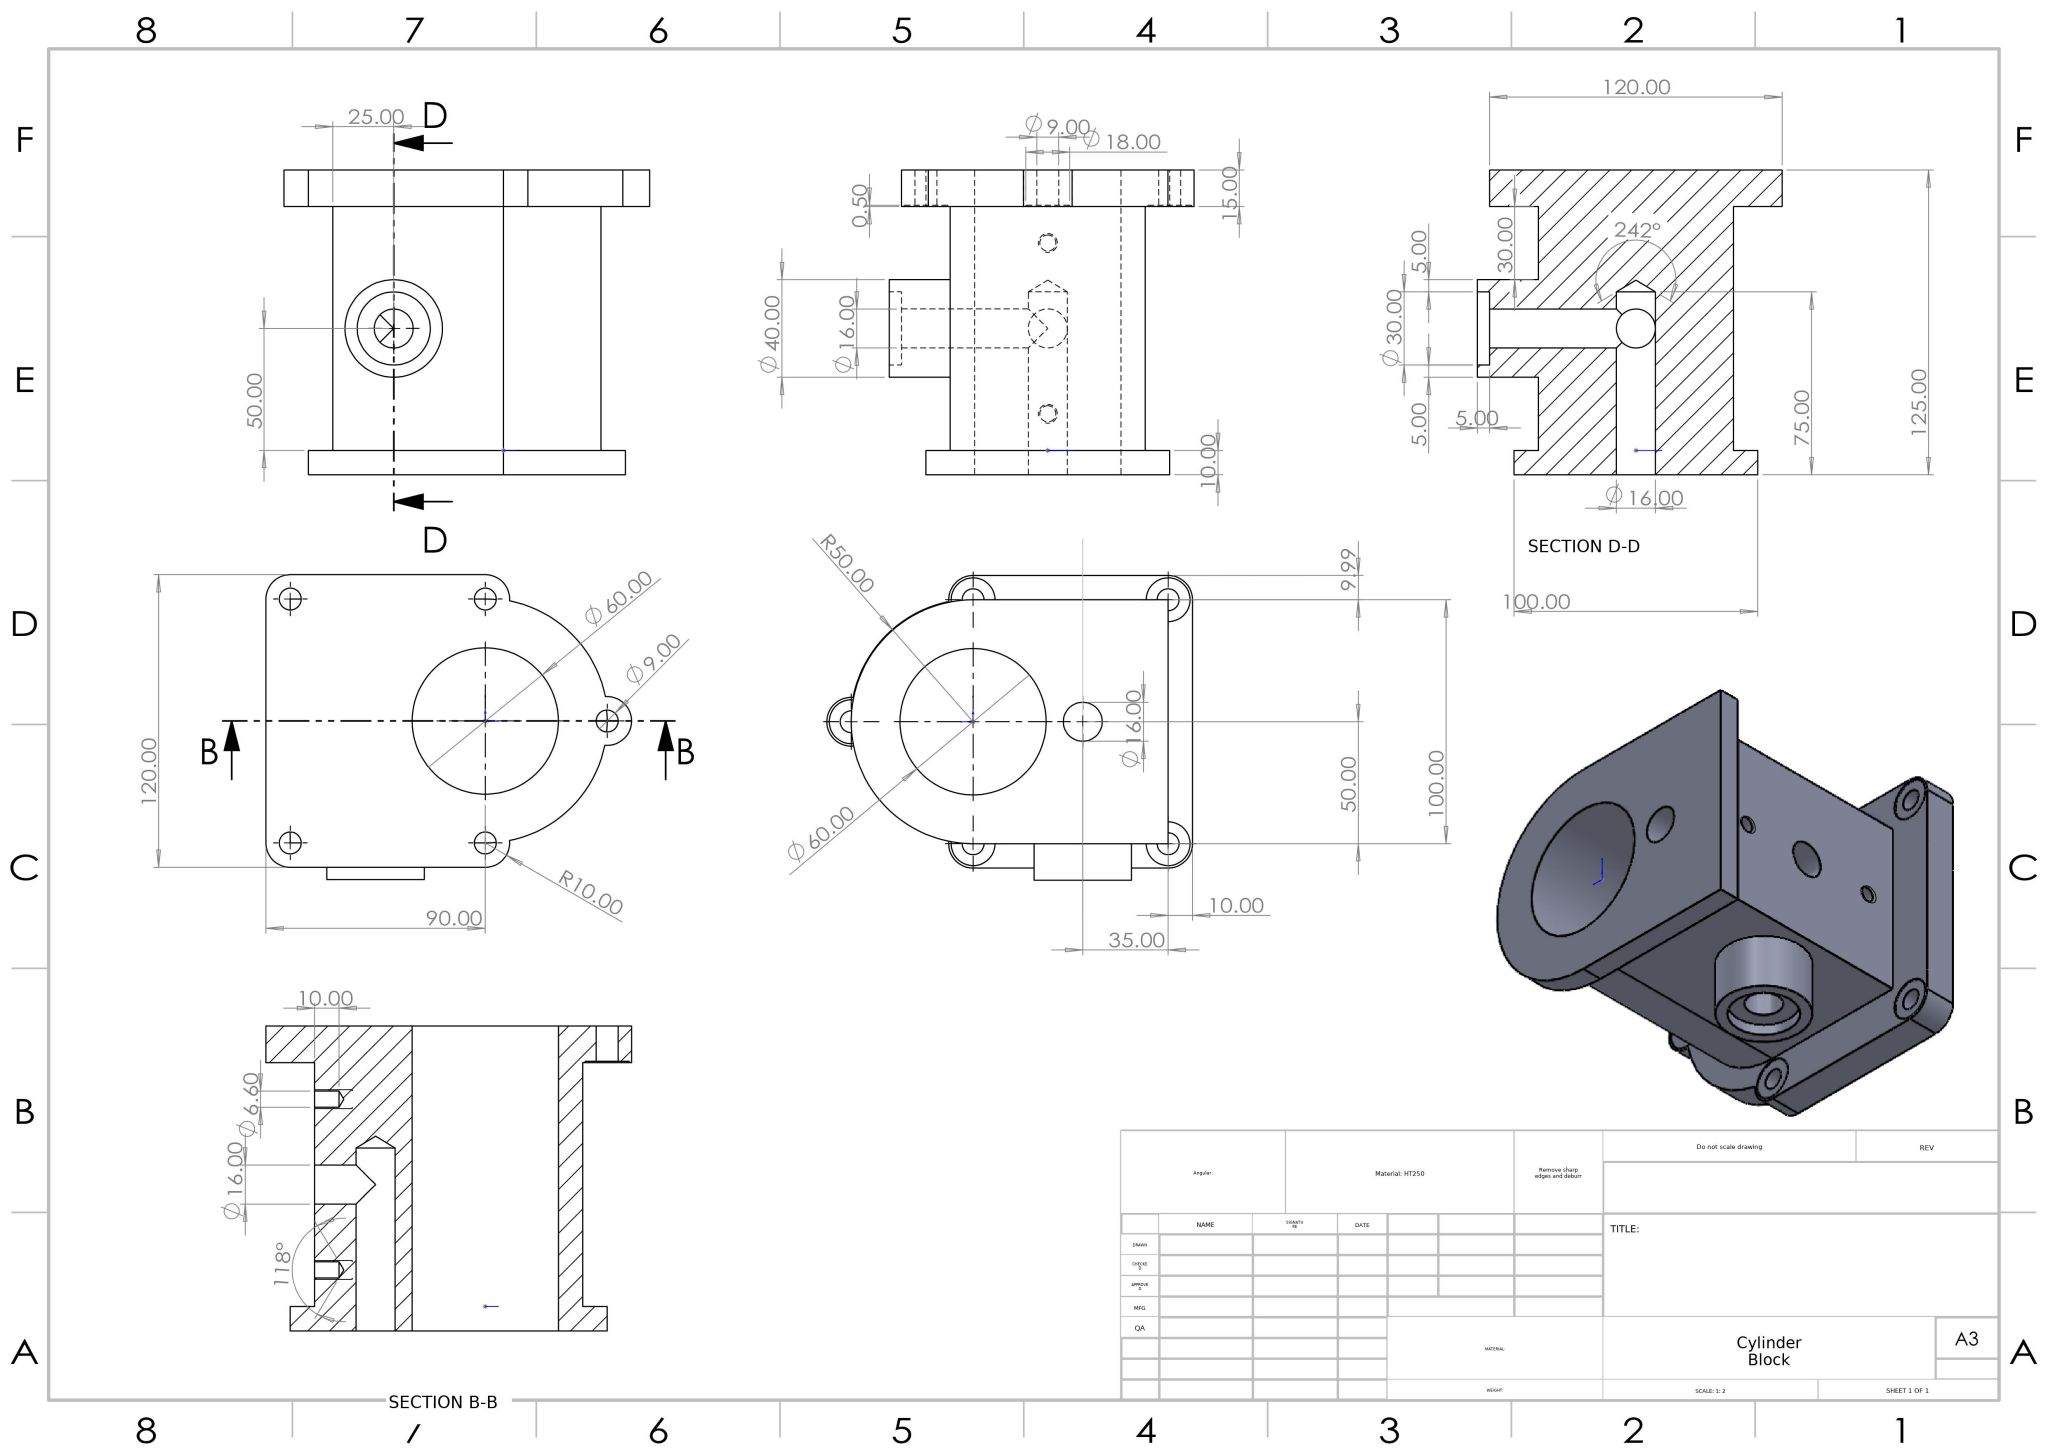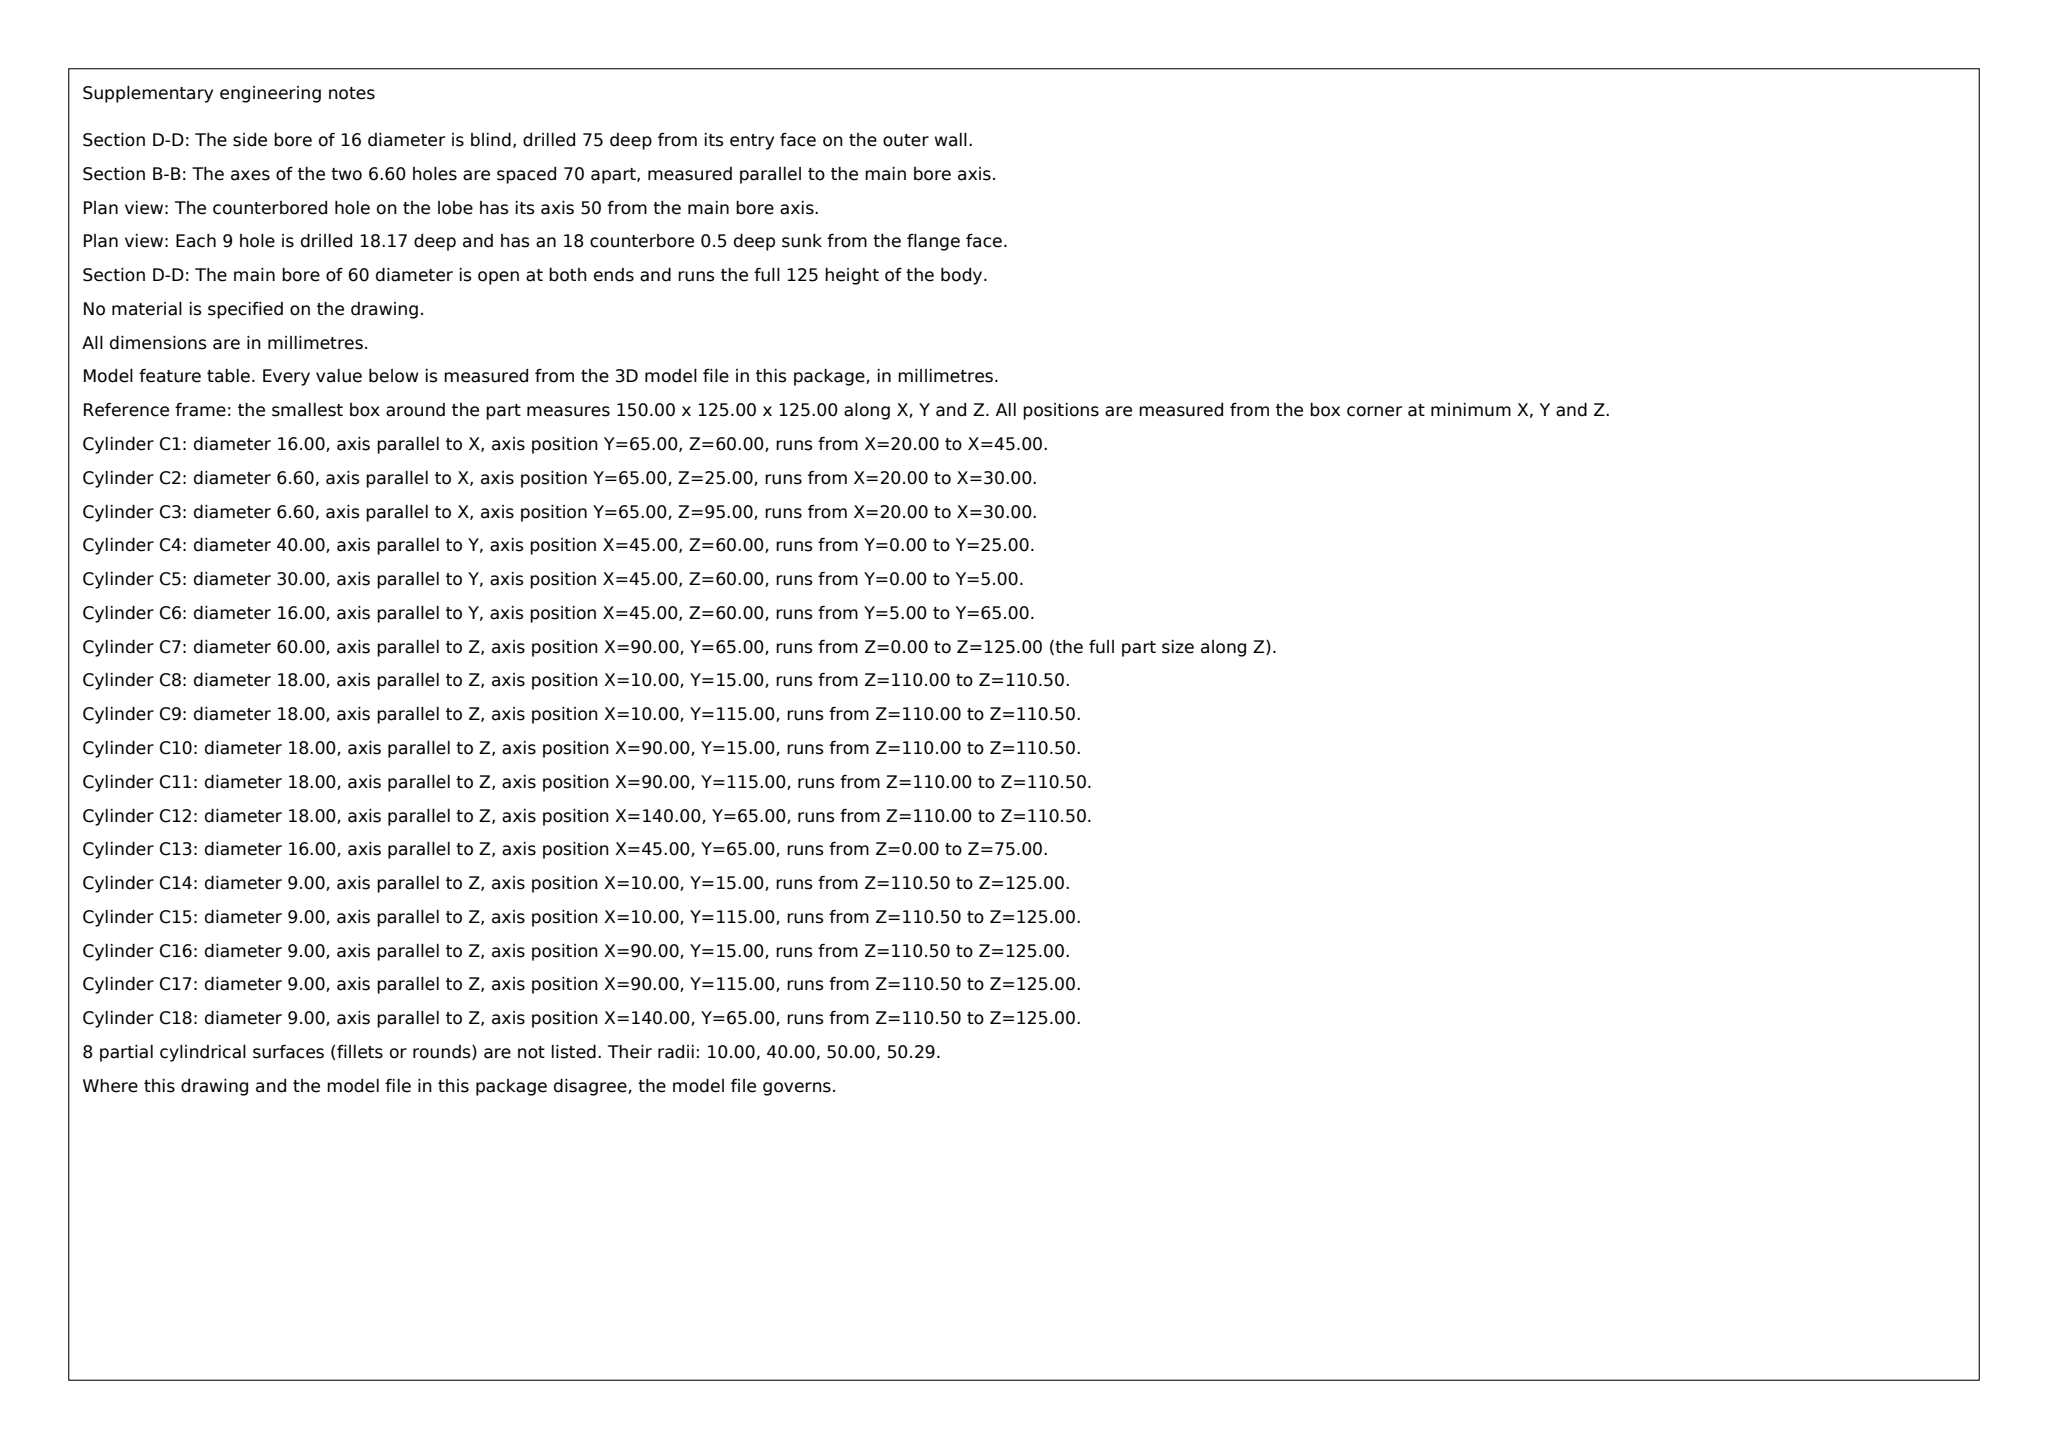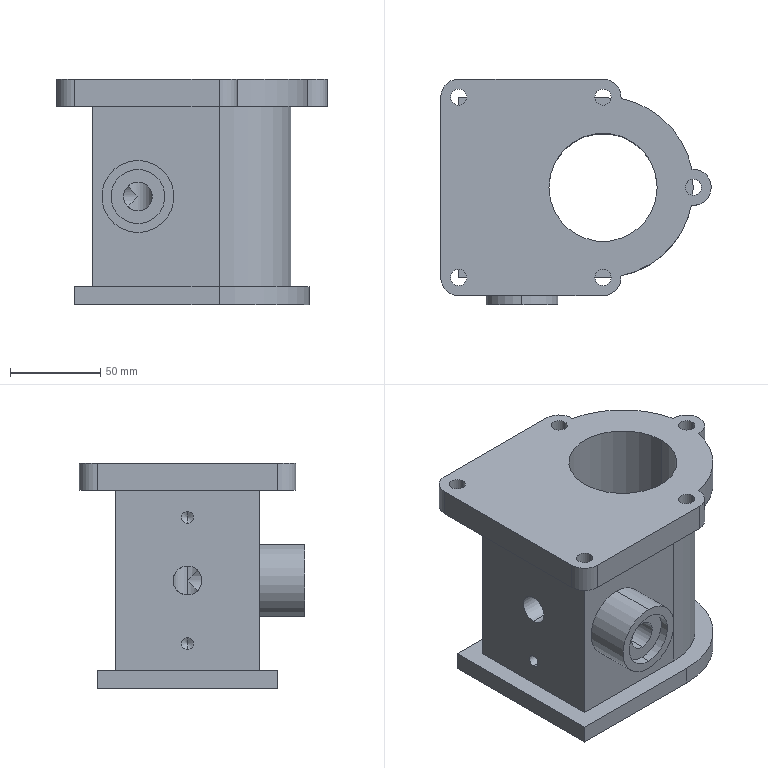Part | SolidWorks | mm | 1 solid | 73 faces | box 150 x 125 x 125 mm | volume 794820 mm3 | cylinder 47 | plane 20 | cone 6 | commonest cylinder face diameters 18 x10 9 x10 16 x7 20 x5 6.6 x4 100 x3 30 x2 40 x2
Drawing notes:
CENTRAL BODY OD Ø80, 100 LG BTWN Ø100 FLANGES | from the solid: cyl [80,"z",[90,65],100] between Ø100 flanges at z0-10 and z110-125
4X Ø6.60 DP 10 (118° PT): CL 25 & 95 FROM BASE, SECT B-B | from the solid: cyls [6.6,"x",[null,65,25],10,2] and [6.6,"x",[null,65,95],10,2]; cones 118°/6.6
SECT B-B: Ø16 BLIND HOLE DP 25 FROM O/S FACE, 118° PT | from the solid: cyl [16,'x',[null,65,60],25.0] with cone 118°, ref_dia 16
ARM Ø16 BORE DP 60 FROM Ø40/Ø30 BOSS END FACE | from the solid: cyl [16,'y',[45,null,60],60.0]; Ø40 L25 & Ø30 L5 boss on same axis
4X Ø6.60 DP 10 118° PT ALL ON CL B-B (Y=65), 2 EA AT 25 & 95 | from the solid: cyls [6.6,'x',[null,65,25],10]x2 and [6.6,'x',[null,65,95],10]x2; 4 cones 118° ref 6.6
SIDE LUG: Ø9 THRU ON Ø20 BOSS, Ø18 SPOTFACE DP 0.50; LUG AXIS AT X=140 FROM PLATE O/S FACE (X=0), Y=65 (PART C/L) | from the solid: cylinders dia 9 (L14.5), dia 18 (L0.5) and dia 20 (L15), axis z, pos [140.0, 65.0]
OVERALL ENVELOPE 150 (X) X 125 (Y) X 125 (Z); X=150 MEASURED FROM PLATE O/S FACE TO SIDE-LUG BOSS O/S | from the solid: bbox_xyz [150.0, 125.0, 125.0]
ARM BOSS: Ø30 X 5 LG FROM END FACE Y=0, THEN Ø40 X 25 LG (ARM PROJECTS 30 TOTAL FROM Y=0); ARM AXIS X=45, Z=60 | from the solid: cylinders dia 30 axis y [45.0,60.0] L5.0 and dia 40 axis y [45.0,60.0] L25.0; planes y=0.0, y=5.0, y=25.0
VERTICAL Ø16 BLIND HOLE DP 75 FROM BASE (Z=0), 118° PT, AXIS AT X=45, Y=65 | from the solid: cylinder dia 16 axis z pos [45.0,65.0] length 75.0; cones 118.0 ref_dia 16.0
4X Ø6.60 DP 10, 118° PT: holes on part C/L Y=65 at Z=25 & 95, axes parallel to X, drilled DP 10 from plate O/S face X=0. | from the solid: cylinders [6.6,"x",[null,65,25],10,2] and [6.6,"x",[null,65,95],10,2]; axis_plane x=0; cones 118° ref dia 6.6 (4)
SIDE LUG: Ø9 THRU on Ø20 boss (boss 15 LG), Ø18 SPOTFACE DP 0.50; lug axis at X=140 from plate O/S face (X=0) and Y=65 (part C/L). | from the solid: cylinders [9.0,"z",[140,65,null],14.5,2], [18.0,"z",[140,65,null],0.5,2], [20.0,"z",[140,65,null],15.0,1]
OVERALL ENVELOPE 150 (X) X 125 (Y) X 125 (Z); X=150 from plate O/S face (X=0) to side-lug boss O/S. | from the solid: bbox_xyz [150.0,125.0,125.0]
ARM BOSS: Ø30 X 5 LG from end face Y=0, then Ø40 X 25 LG (arm projects 30 total from Y=0); arm axis at X=45, Z=60. | from the solid: cylinders [30.0,"y",[45,null,60],5.0,2] and [40.0,"y",[45,null,60],25.0,2]; axis_planes y=0, y=5, y=25
VERTICAL Ø16 BLIND HOLE DP 75 FROM BASE (Z=0), 118° PT; axis at X=45, Y=65. | from the solid: cylinder [16.0,"z",[45,65,null],75.0,1]; cones 118° ref dia 16 (2); axis_plane z=0
build123d program:
from build123d import *

# Parameters (mm, degrees)
SKETCH1_5_R                                         = 30
BOSS_EXTRUDE1_DEPTH                                 = 100
BOSS_EXTRUDE2_START                                 = -10
SKETCH1_4_R                                         = 30
BOSS_EXTRUDE2_DEPTH                                 = 10
F_16_0_16_DIAMETER_HOLE1_D                          = 16
F_16_0_16_DIAMETER_HOLE1_DEPTH                      = 75
F_16_0_16_DIAMETER_HOLE1_TIP                        = 4.807
CUT_EXTRUDE1_DEPTH                                  = 40
SKETCH4_R                                           = 8
CUT_EXTRUDE2_DEPTH                                  = 25
BOSS_EXTRUDE3_START                                 = 20
BOSS_EXTRUDE3_DEPTH                                 = 20
BOSS_EXTRUDE4_START                                 = 25
BOSS_EXTRUDE4_DEPTH                                 = 25
G1_16_TAPPED_HOLE1_D                                = 6.6
G1_16_TAPPED_HOLE1_DEPTH                            = 10
G1_16_TAPPED_HOLE1_TIP                              = 1.983
CUT_EXTRUDE4_START                                  = -25
SKETCH1_5_2_R                                       = 30
CUT_EXTRUDE4_DEPTH                                  = 25
SKETCH10_R                                          = 30
BOSS_EXTRUDE5_DEPTH                                 = 15
CYLINDRICAL_COUNTERSUNK_HOLE_FOR_M8_HEX_D           = 9
CYLINDRICAL_COUNTERSUNK_HOLE_FOR_M8_HEX_DEPTH       = 18.17
CYLINDRICAL_COUNTERSUNK_HOLE_FOR_M8_HEX_CBORE_D     = 18
CYLINDRICAL_COUNTERSUNK_HOLE_FOR_M8_HEX_CBORE_DEPTH = 0.5
CYLINDRICAL_COUNTERSUNK_HOLE_FOR_M8_HEX_TIP         = 2.704


with BuildPart() as part:
    # Sketch1_5 → Boss-Extrude1 (new body)
    # profile 1 of 2: a face of its own
    with BuildSketch(Plane.XY):
        with BuildLine():
            ThreePointArc((0, 40), (-40, 0), (0, -40))
            Line((0, -40), (-70, -40))
            Line((-70, -40), (-70, 40))
            Line((-70, 40), (0, 40))
        make_face()
    # profile 2 of 2: a face of its own
    with BuildSketch(Plane.XY):
        with BuildLine():
            ThreePointArc((0, 40), (40, 0), (0, -40))
            ThreePointArc((0, -40), (-40, 0), (0, 40))
        make_face()
        Circle(SKETCH1_5_R, mode=Mode.SUBTRACT)
    extrude(amount=BOSS_EXTRUDE1_DEPTH)

    # Sketch1_4 → Boss-Extrude2 (add)
    # profile 1 of 4: a face of its own
    with BuildSketch(Plane.XY.offset(BOSS_EXTRUDE2_START)):
        with BuildLine():
            ThreePointArc((0, 50), (50, 0), (0, -50))
            Line((0, -50), (-80, -50))
            Line((-80, -50), (-80, 50))
            Line((-80, 50), (0, 50))
        make_face()
        with BuildLine():
            Line((-70, 40), (0, 40))
            ThreePointArc((0, 40), (40, 0), (0, -40))
            Line((0, -40), (-70, -40))
            Line((-70, -40), (-70, 40))
        make_face(mode=Mode.SUBTRACT)
    # profile 2 of 4: a face of its own
    with BuildSketch(Plane.XY.offset(BOSS_EXTRUDE2_START)):
        with BuildLine():
            ThreePointArc((0, 40), (40, 0), (0, -40))
            ThreePointArc((0, -40), (-40, 0), (0, 40))
        make_face()
        Circle(SKETCH1_4_R, mode=Mode.SUBTRACT)
    # profile 3 of 4: a face of its own
    with BuildSketch(Plane.XY.offset(BOSS_EXTRUDE2_START)):
        Circle(SKETCH1_4_R)
    # profile 4 of 4: a face of its own
    with BuildSketch(Plane.XY.offset(BOSS_EXTRUDE2_START)):
        with BuildLine():
            ThreePointArc((0, 40), (-40, 0), (0, -40))
            Line((0, -40), (-70, -40))
            Line((-70, -40), (-70, 40))
            Line((-70, 40), (0, 40))
        make_face()
    extrude(amount=BOSS_EXTRUDE2_DEPTH)

    # 16.0 _16_ Diameter Hole1
    with Locations(Plane(origin=(0, 0, -10), x_dir=(-1, 0, 0), z_dir=(0, 0, -1))):
        with Locations((45, 0)):
            Hole(F_16_0_16_DIAMETER_HOLE1_D / 2, depth=F_16_0_16_DIAMETER_HOLE1_DEPTH)
            with Locations((0, 0, -(F_16_0_16_DIAMETER_HOLE1_DEPTH + F_16_0_16_DIAMETER_HOLE1_TIP / 2))):  # 118° drill point
                Cone(0, F_16_0_16_DIAMETER_HOLE1_D / 2, F_16_0_16_DIAMETER_HOLE1_TIP, mode=Mode.SUBTRACT)

    # Sketch5_5 → Cut-Extrude1 (cut)
    with BuildSketch(Plane.XZ.offset(40)):
        with BuildLine():
            ThreePointArc((-45, 58), (-53, 50), (-45, 42))
            Line((-45, 42), (-45, 58))
        make_face()
        with BuildLine():
            Line((-45, 58), (-45, 42))
            ThreePointArc((-45, 42), (-39.343, 44.343), (-37, 50))
            ThreePointArc((-37, 50), (-39.343, 55.657), (-45, 58))
        make_face()
        with BuildLine():
            ThreePointArc((-45, 58), (-53, 50), (-45, 42))
            Line((-45, 42), (-45, 58))
        make_face()
        with BuildLine():
            Line((-45, 58), (-45, 42))
            ThreePointArc((-45, 42), (-39.343, 44.343), (-37, 50))
            ThreePointArc((-37, 50), (-39.343, 55.657), (-45, 58))
        make_face()
    extrude(amount=-CUT_EXTRUDE1_DEPTH, mode=Mode.SUBTRACT)

    # Sketch4 → Cut-Extrude2 (cut)
    with BuildSketch(Plane.ZY.offset(70)):
        with Locations((50, 0)):
            Circle(SKETCH4_R)
    extrude(amount=-CUT_EXTRUDE2_DEPTH, mode=Mode.SUBTRACT)

    # Sketch5_4 → Boss-Extrude3 (add)
    with BuildSketch(Plane.XZ.offset(40).offset(BOSS_EXTRUDE3_START)):
        with BuildLine():
            ThreePointArc((-45, 65), (-60, 50), (-45, 35))
            Line((-45, 35), (-45, 42))
            ThreePointArc((-45, 42), (-53, 50), (-45, 58))
            Line((-45, 58), (-45, 65))
        make_face()
        with BuildLine():
            Line((-45, 42), (-45, 35))
            ThreePointArc((-45, 35), (-34.393, 39.393), (-30, 50))
            ThreePointArc((-30, 50), (-34.393, 60.607), (-45, 65))
            Line((-45, 65), (-45, 58))
            ThreePointArc((-45, 58), (-39.343, 55.657), (-37, 50))
            ThreePointArc((-37, 50), (-39.343, 44.343), (-45, 42))
        make_face()
        with BuildLine():
            ThreePointArc((-45, 65), (-60, 50), (-45, 35))
            Line((-45, 35), (-45, 42))
            ThreePointArc((-45, 42), (-53, 50), (-45, 58))
            Line((-45, 58), (-45, 65))
        make_face()
        with BuildLine():
            Line((-45, 42), (-45, 35))
            ThreePointArc((-45, 35), (-34.393, 39.393), (-30, 50))
            ThreePointArc((-30, 50), (-34.393, 60.607), (-45, 65))
            Line((-45, 65), (-45, 58))
            ThreePointArc((-45, 58), (-39.343, 55.657), (-37, 50))
            ThreePointArc((-37, 50), (-39.343, 44.343), (-45, 42))
        make_face()
        with BuildLine():
            ThreePointArc((-45, 70), (-65, 50), (-45, 30))
            Line((-45, 30), (-45, 35))
            ThreePointArc((-45, 35), (-60, 50), (-45, 65))
            Line((-45, 65), (-45, 70))
        make_face()
        with BuildLine():
            Line((-45, 35), (-45, 30))
            ThreePointArc((-45, 30), (-30.858, 35.858), (-25, 50))
            ThreePointArc((-25, 50), (-30.858, 64.142), (-45, 70))
            Line((-45, 70), (-45, 65))
            ThreePointArc((-45, 65), (-34.393, 60.607), (-30, 50))
            ThreePointArc((-30, 50), (-34.393, 39.393), (-45, 35))
        make_face()
        with BuildLine():
            ThreePointArc((-45, 70), (-65, 50), (-45, 30))
            Line((-45, 30), (-45, 35))
            ThreePointArc((-45, 35), (-60, 50), (-45, 65))
            Line((-45, 65), (-45, 70))
        make_face()
        with BuildLine():
            Line((-45, 35), (-45, 30))
            ThreePointArc((-45, 30), (-30.858, 35.858), (-25, 50))
            ThreePointArc((-25, 50), (-30.858, 64.142), (-45, 70))
            Line((-45, 70), (-45, 65))
            ThreePointArc((-45, 65), (-34.393, 60.607), (-30, 50))
            ThreePointArc((-30, 50), (-34.393, 39.393), (-45, 35))
        make_face()
    extrude(amount=-BOSS_EXTRUDE3_DEPTH)

    # Sketch5_5 2 → Boss-Extrude4 (add)
    with BuildSketch(Plane.XZ.offset(40).offset(BOSS_EXTRUDE4_START)):
        with BuildLine():
            ThreePointArc((-45, 70), (-65, 50), (-45, 30))
            Line((-45, 30), (-45, 35))
            ThreePointArc((-45, 35), (-60, 50), (-45, 65))
            Line((-45, 65), (-45, 70))
        make_face()
        with BuildLine():
            Line((-45, 35), (-45, 30))
            ThreePointArc((-45, 30), (-30.858, 35.858), (-25, 50))
            ThreePointArc((-25, 50), (-30.858, 64.142), (-45, 70))
            Line((-45, 70), (-45, 65))
            ThreePointArc((-45, 65), (-34.393, 60.607), (-30, 50))
            ThreePointArc((-30, 50), (-34.393, 39.393), (-45, 35))
        make_face()
        with BuildLine():
            ThreePointArc((-45, 70), (-65, 50), (-45, 30))
            Line((-45, 30), (-45, 35))
            ThreePointArc((-45, 35), (-60, 50), (-45, 65))
            Line((-45, 65), (-45, 70))
        make_face()
        with BuildLine():
            Line((-45, 35), (-45, 30))
            ThreePointArc((-45, 30), (-30.858, 35.858), (-25, 50))
            ThreePointArc((-25, 50), (-30.858, 64.142), (-45, 70))
            Line((-45, 70), (-45, 65))
            ThreePointArc((-45, 65), (-34.393, 60.607), (-30, 50))
            ThreePointArc((-30, 50), (-34.393, 39.393), (-45, 35))
        make_face()
    extrude(amount=-BOSS_EXTRUDE4_DEPTH)

    # G1_16 Tapped Hole1
    with Locations(Plane(origin=(-70, 0, 85), x_dir=(0, 0, -1), z_dir=(-1, 0, 0))):
        with Locations((0, 0), (70, 0)):
            Hole(G1_16_TAPPED_HOLE1_D / 2, depth=G1_16_TAPPED_HOLE1_DEPTH)
            with Locations((0, 0, -(G1_16_TAPPED_HOLE1_DEPTH + G1_16_TAPPED_HOLE1_TIP / 2))):  # 118° drill point
                Cone(0, G1_16_TAPPED_HOLE1_D / 2, G1_16_TAPPED_HOLE1_TIP, mode=Mode.SUBTRACT)

    # Sketch1_5 2 → Cut-Extrude4 (cut)
    with BuildSketch(Plane.XY.offset(CUT_EXTRUDE4_START)):
        Circle(SKETCH1_5_2_R)
    extrude(amount=CUT_EXTRUDE4_DEPTH, mode=Mode.SUBTRACT)

    # Sketch10 → Boss-Extrude5 (add)
    # profile 1 of 2: a face of its own
    with BuildSketch(Plane.XY.offset(100)):
        with BuildLine():
            Line((-90, 50), (-90, -50))
            ThreePointArc((-90, -50), (-87.071, -57.071), (-80, -60))
            Line((-80, -60), (0, -60))
            ThreePointArc((0, -60), (7.416, -56.708), (9.95, -49))
            ThreePointArc((9.95, -49), (35.355, -35.355), (49, -9.95))
            ThreePointArc((49, -9.95), (59.999, -0.147), (49.293, 9.975))
            ThreePointArc((49.293, 9.975), (35.562, 35.562), (9.975, 49.293))
            ThreePointArc((9.975, 49.293), (7.436, 56.686), (0.3537, 59.994))
            Line((0.3537, 59.994), (-0.3522, 59.994))
            Line((-0.3522, 59.994), (-79.998, 60))
            Line((-79.998, 60), (-80, 60))
            ThreePointArc((-80, 60), (-87.071, 57.071), (-90, 50))
        make_face()
        with BuildLine():
            Line((0, -40), (-70, -40))
            Line((-70, -40), (-70, 40))
            Line((-70, 40), (0, 40))
            ThreePointArc((0, 40), (40, 0), (0, -40))
        make_face(mode=Mode.SUBTRACT)
    # profile 2 of 2: a face of its own
    with BuildSketch(Plane.XY.offset(100)):
        with BuildLine():
            Line((-70, 40), (-70, -40))
            Line((-70, -40), (0, -40))
            ThreePointArc((0, -40), (40, 0), (0, 40))
            Line((0, 40), (-70, 40))
        make_face()
        Circle(SKETCH10_R, mode=Mode.SUBTRACT)
    extrude(amount=BOSS_EXTRUDE5_DEPTH)

    # Cylindrical Countersunk Hole for M8 Hex
    with Locations(Plane(origin=(0, 0, 100), x_dir=(-1, 0, 0), z_dir=(0, 0, -1))):
        with Locations((-50, 0), (0, -50), (80, -50), (80, 50), (0, 50)):
            CounterBoreHole(CYLINDRICAL_COUNTERSUNK_HOLE_FOR_M8_HEX_D / 2, CYLINDRICAL_COUNTERSUNK_HOLE_FOR_M8_HEX_CBORE_D / 2, CYLINDRICAL_COUNTERSUNK_HOLE_FOR_M8_HEX_CBORE_DEPTH, depth=CYLINDRICAL_COUNTERSUNK_HOLE_FOR_M8_HEX_DEPTH)
            with Locations((0, 0, -(CYLINDRICAL_COUNTERSUNK_HOLE_FOR_M8_HEX_DEPTH + CYLINDRICAL_COUNTERSUNK_HOLE_FOR_M8_HEX_TIP / 2))):  # 118° drill point
                Cone(0, CYLINDRICAL_COUNTERSUNK_HOLE_FOR_M8_HEX_D / 2, CYLINDRICAL_COUNTERSUNK_HOLE_FOR_M8_HEX_TIP, mode=Mode.SUBTRACT)


solid = part.part